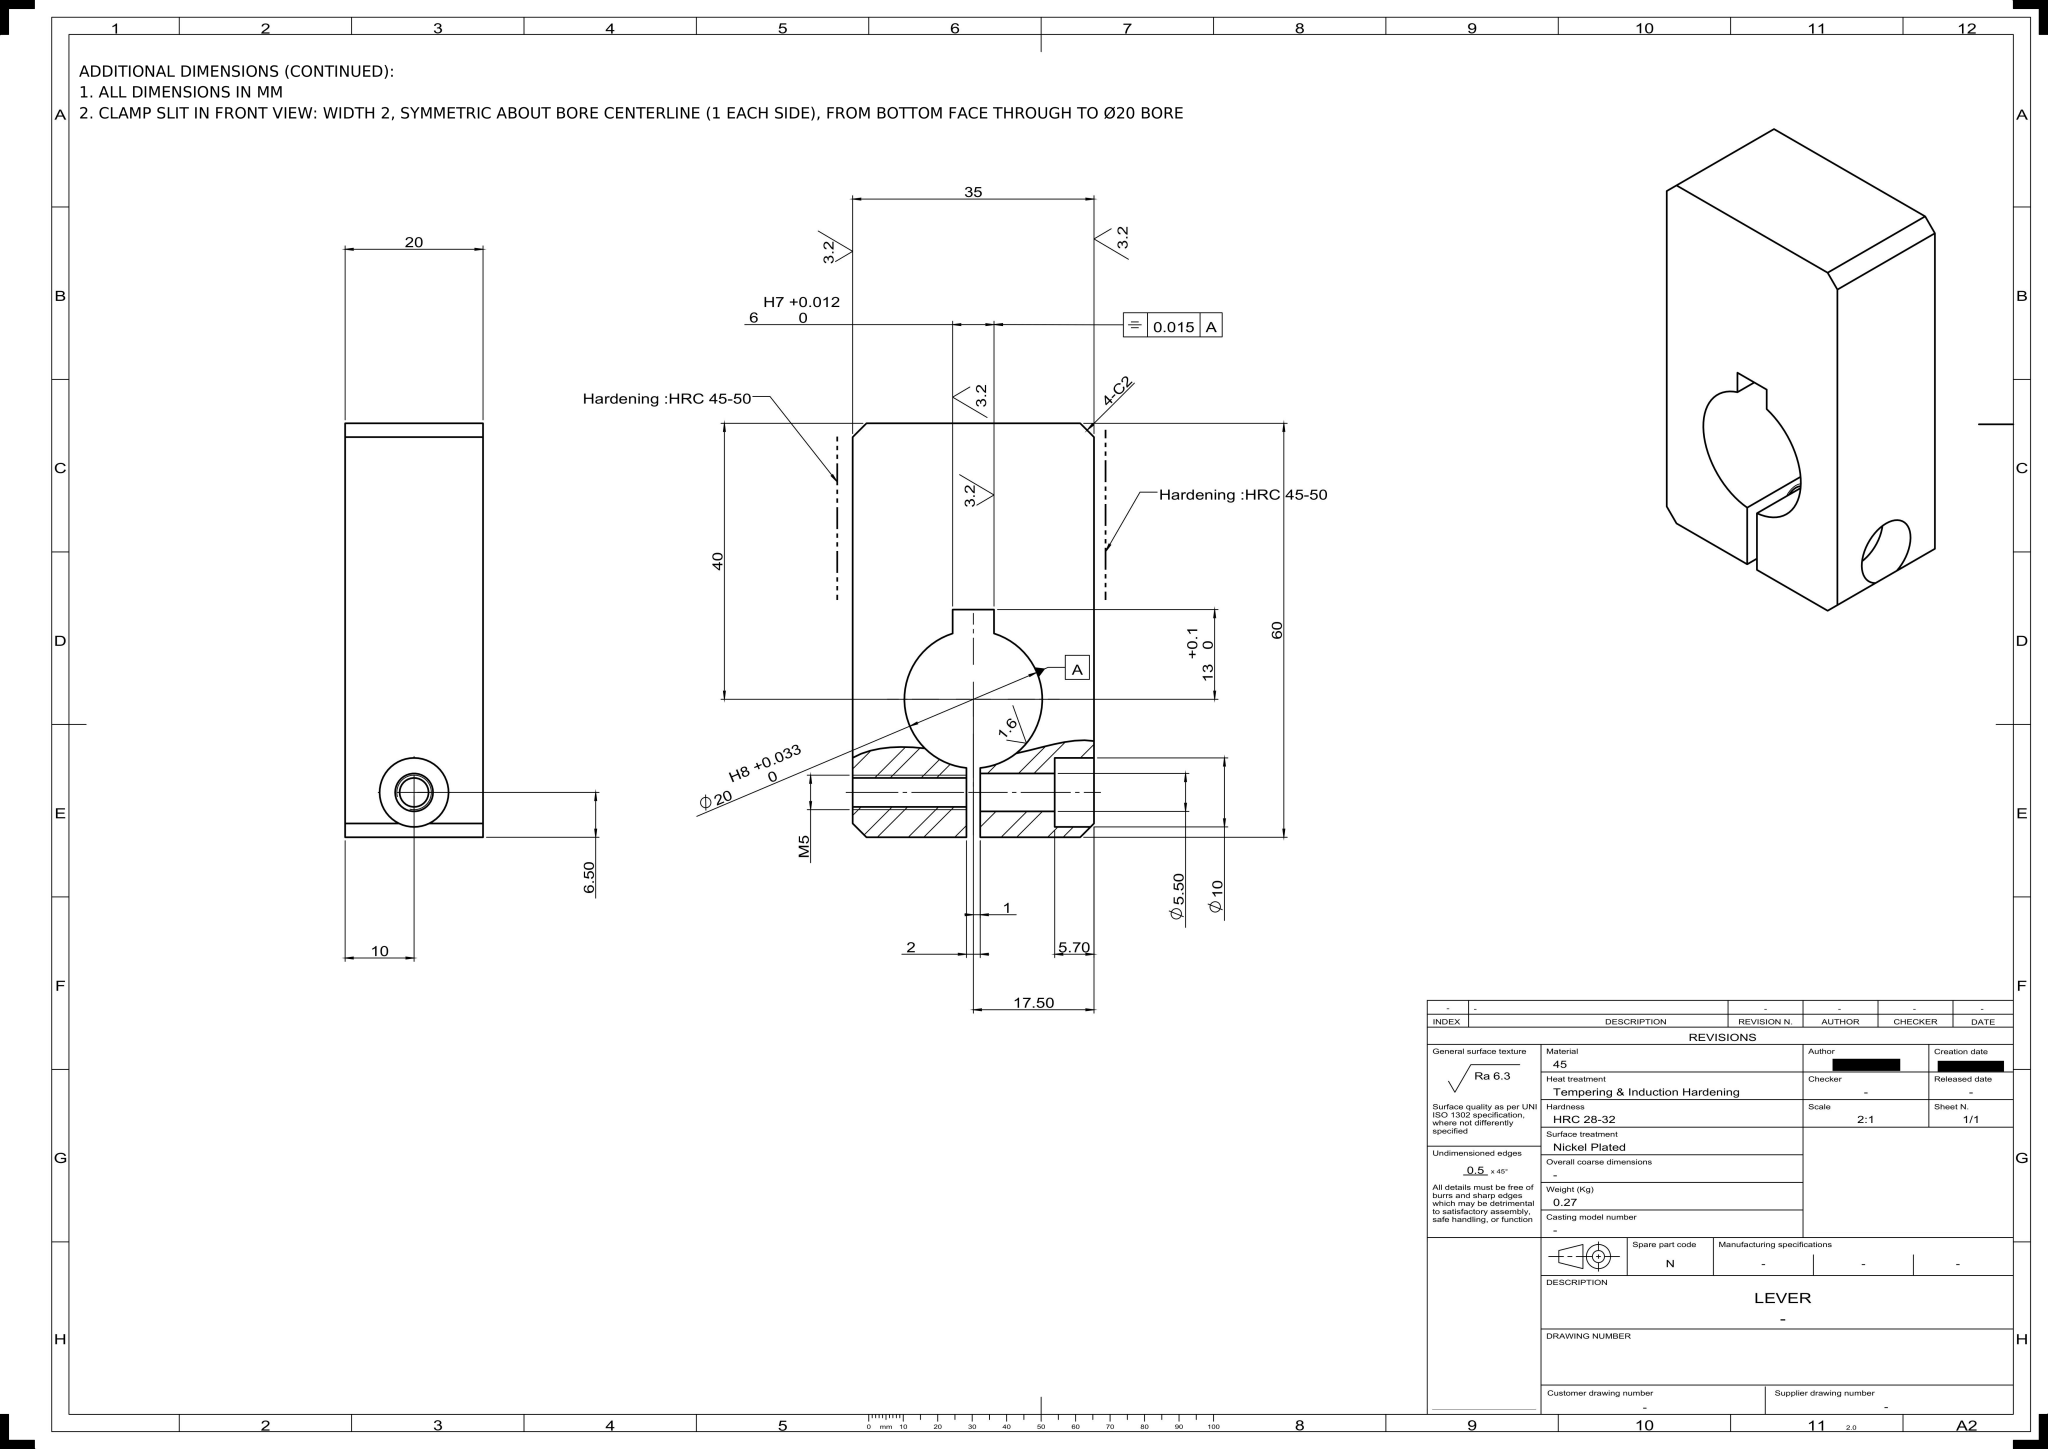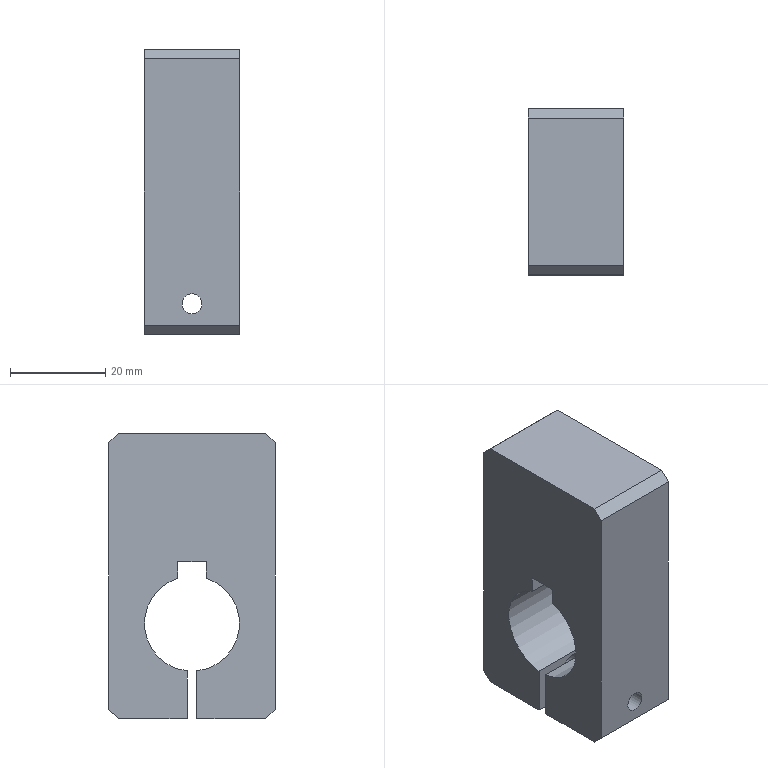Part | NX | mm | 1 solid | 22 faces | box 20 x 35 x 60 mm | volume 33845 mm3 | plane 17 | cylinder 5 | commonest cylinder face diameters 20 x2 5.5 x1 10 x1 4.2 x1
STEP:
#1=CARTESIAN_POINT('',(0.,0.,0.));
#2=DIRECTION('',(0.,0.,1.));
#3=DIRECTION('',(1.,0.,0.));
#4=AXIS2_PLACEMENT_3D('',#1,#2,#3);
#5=(LENGTH_UNIT()NAMED_UNIT(*)SI_UNIT(.MILLI.,.METRE.));
#6=UNCERTAINTY_MEASURE_WITH_UNIT(LENGTH_MEASURE(0.00002),#5,'','');
#7=(NAMED_UNIT(*)PLANE_ANGLE_UNIT()SI_UNIT($,.RADIAN.));
#8=PLANE_ANGLE_MEASURE_WITH_UNIT(PLANE_ANGLE_MEASURE(0.01745),#7);
#9=DIMENSIONAL_EXPONENTS(0.,0.,0.,0.,0.,0.,0.);
#10=(CONVERSION_BASED_UNIT('',#8)NAMED_UNIT(#9)PLANE_ANGLE_UNIT());
#11=(NAMED_UNIT(*)SI_UNIT($,.STERADIAN.)SOLID_ANGLE_UNIT());
#12=(GEOMETRIC_REPRESENTATION_CONTEXT(3)GLOBAL_UNCERTAINTY_ASSIGNED_CONTEXT((#6))GLOBAL_UNIT_ASSIGNED_CONTEXT((#5,#10,#11))REPRESENTATION_CONTEXT('',''));
#13=SHAPE_REPRESENTATION('',(#4),#12);
#14=CARTESIAN_POINT('',(10.,17.5,-18.));
#15=VERTEX_POINT('',#14);
#16=CARTESIAN_POINT('',(10.,17.5,38.));
#17=VERTEX_POINT('',#16);
#18=CARTESIAN_POINT('',(10.,17.5,-20.));
#19=DIRECTION('',(0.,0.,1.));
#20=VECTOR('',#19,1.);
#21=LINE('',#18,#20);
#22=EDGE_CURVE('',#15,#17,#21,.T.);
#23=ORIENTED_EDGE('',*,*,#22,.T.);
#24=CARTESIAN_POINT('',(10.,15.5,40.));
#25=VERTEX_POINT('',#24);
#26=CARTESIAN_POINT('',(10.,27.75,27.75));
#27=DIRECTION('',(0.,-0.7071,0.7071));
#28=VECTOR('',#27,1.);
#29=LINE('',#26,#28);
#30=EDGE_CURVE('',#17,#25,#29,.T.);
#31=ORIENTED_EDGE('',*,*,#30,.T.);
#32=CARTESIAN_POINT('',(10.,-15.5,40.));
#33=VERTEX_POINT('',#32);
#34=CARTESIAN_POINT('',(10.,17.5,40.));
#35=DIRECTION('',(0.,-1.,0.));
#36=VECTOR('',#35,1.);
#37=LINE('',#34,#36);
#38=EDGE_CURVE('',#25,#33,#37,.T.);
#39=ORIENTED_EDGE('',*,*,#38,.T.);
#40=CARTESIAN_POINT('',(10.,-17.5,38.));
#41=VERTEX_POINT('',#40);
#42=CARTESIAN_POINT('',(10.,-27.75,27.75));
#43=DIRECTION('',(0.,-0.7071,-0.7071));
#44=VECTOR('',#43,1.);
#45=LINE('',#42,#44);
#46=EDGE_CURVE('',#33,#41,#45,.T.);
#47=ORIENTED_EDGE('',*,*,#46,.T.);
#48=CARTESIAN_POINT('',(10.,-17.5,-18.));
#49=VERTEX_POINT('',#48);
#50=CARTESIAN_POINT('',(10.,-17.5,40.));
#51=DIRECTION('',(0.,0.,-1.));
#52=VECTOR('',#51,1.);
#53=LINE('',#50,#52);
#54=EDGE_CURVE('',#41,#49,#53,.T.);
#55=ORIENTED_EDGE('',*,*,#54,.T.);
#56=CARTESIAN_POINT('',(10.,-15.5,-20.));
#57=VERTEX_POINT('',#56);
#58=CARTESIAN_POINT('',(10.,-17.75,-17.75));
#59=DIRECTION('',(0.,0.7071,-0.7071));
#60=VECTOR('',#59,1.);
#61=LINE('',#58,#60);
#62=EDGE_CURVE('',#49,#57,#61,.T.);
#63=ORIENTED_EDGE('',*,*,#62,.T.);
#64=CARTESIAN_POINT('',(10.,-1.,-20.));
#65=VERTEX_POINT('',#64);
#66=CARTESIAN_POINT('',(10.,-17.5,-20.));
#67=DIRECTION('',(0.,1.,0.));
#68=VECTOR('',#67,1.);
#69=LINE('',#66,#68);
#70=EDGE_CURVE('',#57,#65,#69,.T.);
#71=ORIENTED_EDGE('',*,*,#70,.T.);
#72=CARTESIAN_POINT('',(10.,-1.,-9.95));
#73=VERTEX_POINT('',#72);
#74=CARTESIAN_POINT('',(10.,-1.,-20.));
#75=DIRECTION('',(0.,0.,1.));
#76=VECTOR('',#75,1.);
#77=LINE('',#74,#76);
#78=EDGE_CURVE('',#65,#73,#77,.T.);
#79=ORIENTED_EDGE('',*,*,#78,.T.);
#80=CARTESIAN_POINT('',(10.,-3.,9.539));
#81=VERTEX_POINT('',#80);
#82=CARTESIAN_POINT('',(10.,0.,0.));
#83=DIRECTION('',(-1.,0.,0.));
#84=DIRECTION('',(0.,0.,1.));
#85=AXIS2_PLACEMENT_3D('',#82,#83,#84);
#86=CIRCLE('',#85,10.);
#87=EDGE_CURVE('',#73,#81,#86,.T.);
#88=ORIENTED_EDGE('',*,*,#87,.T.);
#89=CARTESIAN_POINT('',(10.,-3.,13.));
#90=VERTEX_POINT('',#89);
#91=CARTESIAN_POINT('',(10.,-3.,0.));
#92=DIRECTION('',(0.,0.,1.));
#93=VECTOR('',#92,1.);
#94=LINE('',#91,#93);
#95=EDGE_CURVE('',#81,#90,#94,.T.);
#96=ORIENTED_EDGE('',*,*,#95,.T.);
#97=CARTESIAN_POINT('',(10.,3.,13.));
#98=VERTEX_POINT('',#97);
#99=CARTESIAN_POINT('',(10.,-3.,13.));
#100=DIRECTION('',(0.,1.,0.));
#101=VECTOR('',#100,1.);
#102=LINE('',#99,#101);
#103=EDGE_CURVE('',#90,#98,#102,.T.);
#104=ORIENTED_EDGE('',*,*,#103,.T.);
#105=CARTESIAN_POINT('',(10.,3.,9.539));
#106=VERTEX_POINT('',#105);
#107=CARTESIAN_POINT('',(10.,3.,13.));
#108=DIRECTION('',(0.,0.,-1.));
#109=VECTOR('',#108,1.);
#110=LINE('',#107,#109);
#111=EDGE_CURVE('',#98,#106,#110,.T.);
#112=ORIENTED_EDGE('',*,*,#111,.T.);
#113=CARTESIAN_POINT('',(10.,1.,-9.95));
#114=VERTEX_POINT('',#113);
#115=CARTESIAN_POINT('',(10.,0.,0.));
#116=DIRECTION('',(-1.,0.,0.));
#117=DIRECTION('',(0.,0.,1.));
#118=AXIS2_PLACEMENT_3D('',#115,#116,#117);
#119=CIRCLE('',#118,10.);
#120=EDGE_CURVE('',#106,#114,#119,.T.);
#121=ORIENTED_EDGE('',*,*,#120,.T.);
#122=CARTESIAN_POINT('',(10.,1.,-20.));
#123=VERTEX_POINT('',#122);
#124=CARTESIAN_POINT('',(10.,1.,0.));
#125=DIRECTION('',(0.,0.,-1.));
#126=VECTOR('',#125,1.);
#127=LINE('',#124,#126);
#128=EDGE_CURVE('',#114,#123,#127,.T.);
#129=ORIENTED_EDGE('',*,*,#128,.T.);
#130=CARTESIAN_POINT('',(10.,15.5,-20.));
#131=VERTEX_POINT('',#130);
#132=CARTESIAN_POINT('',(10.,1.,-20.));
#133=DIRECTION('',(0.,1.,0.));
#134=VECTOR('',#133,1.);
#135=LINE('',#132,#134);
#136=EDGE_CURVE('',#123,#131,#135,.T.);
#137=ORIENTED_EDGE('',*,*,#136,.T.);
#138=CARTESIAN_POINT('',(10.,17.75,-17.75));
#139=DIRECTION('',(0.,0.7071,0.7071));
#140=VECTOR('',#139,1.);
#141=LINE('',#138,#140);
#142=EDGE_CURVE('',#131,#15,#141,.T.);
#143=ORIENTED_EDGE('',*,*,#142,.T.);
#144=EDGE_LOOP('',(#23,#31,#39,#47,#55,#63,#71,#79,#88,#96,#104,#112,#121,#129,#137,#143));
#145=FACE_OUTER_BOUND('',#144,.T.);
#146=CARTESIAN_POINT('',(10.,0.,0.));
#147=DIRECTION('',(1.,0.,0.));
#148=DIRECTION('',(0.,0.,-1.));
#149=AXIS2_PLACEMENT_3D('',#146,#147,#148);
#150=PLANE('',#149);
#151=ADVANCED_FACE('',(#145),#150,.T.);
#152=CARTESIAN_POINT('',(0.,-17.5,-11.4));
#153=VERTEX_POINT('',#152);
#154=CARTESIAN_POINT('',(0.,-17.5,-13.5));
#155=DIRECTION('',(0.,1.,0.));
#156=DIRECTION('',(0.,0.,1.));
#157=AXIS2_PLACEMENT_3D('',#154,#155,#156);
#158=CIRCLE('',#157,2.1);
#159=EDGE_CURVE('',#153,#153,#158,.T.);
#160=ORIENTED_EDGE('',*,*,#159,.T.);
#161=EDGE_LOOP('',(#160));
#162=FACE_BOUND('',#161,.T.);
#163=ORIENTED_EDGE('',*,*,#54,.F.);
#164=CARTESIAN_POINT('',(-10.,-17.5,38.));
#165=VERTEX_POINT('',#164);
#166=CARTESIAN_POINT('',(10.,-17.5,38.));
#167=DIRECTION('',(-1.,0.,0.));
#168=VECTOR('',#167,1.);
#169=LINE('',#166,#168);
#170=EDGE_CURVE('',#41,#165,#169,.T.);
#171=ORIENTED_EDGE('',*,*,#170,.T.);
#172=CARTESIAN_POINT('',(-10.,-17.5,-18.));
#173=VERTEX_POINT('',#172);
#174=CARTESIAN_POINT('',(-10.,-17.5,40.));
#175=DIRECTION('',(0.,0.,-1.));
#176=VECTOR('',#175,1.);
#177=LINE('',#174,#176);
#178=EDGE_CURVE('',#165,#173,#177,.T.);
#179=ORIENTED_EDGE('',*,*,#178,.T.);
#180=CARTESIAN_POINT('',(10.,-17.5,-18.));
#181=DIRECTION('',(1.,0.,0.));
#182=VECTOR('',#181,1.);
#183=LINE('',#180,#182);
#184=EDGE_CURVE('',#173,#49,#183,.T.);
#185=ORIENTED_EDGE('',*,*,#184,.T.);
#186=EDGE_LOOP('',(#163,#171,#179,#185));
#187=FACE_BOUND('',#186,.T.);
#188=CARTESIAN_POINT('',(10.,-17.5,40.));
#189=DIRECTION('',(0.,1.,0.));
#190=DIRECTION('',(0.,0.,1.));
#191=AXIS2_PLACEMENT_3D('',#188,#189,#190);
#192=PLANE('',#191);
#193=ADVANCED_FACE('',(#162,#187),#192,.F.);
#194=ORIENTED_EDGE('',*,*,#70,.F.);
#195=CARTESIAN_POINT('',(-10.,-15.5,-20.));
#196=VERTEX_POINT('',#195);
#197=CARTESIAN_POINT('',(10.,-15.5,-20.));
#198=DIRECTION('',(-1.,0.,0.));
#199=VECTOR('',#198,1.);
#200=LINE('',#197,#199);
#201=EDGE_CURVE('',#57,#196,#200,.T.);
#202=ORIENTED_EDGE('',*,*,#201,.T.);
#203=CARTESIAN_POINT('',(-10.,-1.,-20.));
#204=VERTEX_POINT('',#203);
#205=CARTESIAN_POINT('',(-10.,-17.5,-20.));
#206=DIRECTION('',(0.,1.,0.));
#207=VECTOR('',#206,1.);
#208=LINE('',#205,#207);
#209=EDGE_CURVE('',#196,#204,#208,.T.);
#210=ORIENTED_EDGE('',*,*,#209,.T.);
#211=CARTESIAN_POINT('',(10.,-1.,-20.));
#212=DIRECTION('',(-1.,0.,0.));
#213=VECTOR('',#212,1.);
#214=LINE('',#211,#213);
#215=EDGE_CURVE('',#65,#204,#214,.T.);
#216=ORIENTED_EDGE('',*,*,#215,.F.);
#217=EDGE_LOOP('',(#194,#202,#210,#216));
#218=FACE_OUTER_BOUND('',#217,.T.);
#219=CARTESIAN_POINT('',(10.,-17.5,-20.));
#220=DIRECTION('',(0.,0.,1.));
#221=DIRECTION('',(1.,0.,0.));
#222=AXIS2_PLACEMENT_3D('',#219,#220,#221);
#223=PLANE('',#222);
#224=ADVANCED_FACE('',(#218),#223,.F.);
#225=CARTESIAN_POINT('',(0.,-1.,-15.6));
#226=VERTEX_POINT('',#225);
#227=CARTESIAN_POINT('',(0.,-1.,-13.5));
#228=DIRECTION('',(0.,-1.,0.));
#229=DIRECTION('',(0.,0.,-1.));
#230=AXIS2_PLACEMENT_3D('',#227,#228,#229);
#231=CIRCLE('',#230,2.1);
#232=EDGE_CURVE('',#226,#226,#231,.T.);
#233=ORIENTED_EDGE('',*,*,#232,.T.);
#234=EDGE_LOOP('',(#233));
#235=FACE_BOUND('',#234,.T.);
#236=CARTESIAN_POINT('',(-10.,-1.,-9.95));
#237=VERTEX_POINT('',#236);
#238=CARTESIAN_POINT('',(-10.,-1.,-20.));
#239=DIRECTION('',(0.,0.,1.));
#240=VECTOR('',#239,1.);
#241=LINE('',#238,#240);
#242=EDGE_CURVE('',#204,#237,#241,.T.);
#243=ORIENTED_EDGE('',*,*,#242,.T.);
#244=CARTESIAN_POINT('',(10.,-1.,-9.95));
#245=DIRECTION('',(1.,0.,0.));
#246=VECTOR('',#245,1.);
#247=LINE('',#244,#246);
#248=EDGE_CURVE('',#237,#73,#247,.T.);
#249=ORIENTED_EDGE('',*,*,#248,.T.);
#250=ORIENTED_EDGE('',*,*,#78,.F.);
#251=ORIENTED_EDGE('',*,*,#215,.T.);
#252=EDGE_LOOP('',(#243,#249,#250,#251));
#253=FACE_BOUND('',#252,.T.);
#254=CARTESIAN_POINT('',(10.,-1.,-20.));
#255=DIRECTION('',(0.,-1.,0.));
#256=DIRECTION('',(0.,0.,-1.));
#257=AXIS2_PLACEMENT_3D('',#254,#255,#256);
#258=PLANE('',#257);
#259=ADVANCED_FACE('',(#235,#253),#258,.F.);
#260=ORIENTED_EDGE('',*,*,#95,.F.);
#261=CARTESIAN_POINT('',(-10.,-3.,9.539));
#262=VERTEX_POINT('',#261);
#263=CARTESIAN_POINT('',(10.,-3.,9.539));
#264=DIRECTION('',(-1.,0.,0.));
#265=VECTOR('',#264,1.);
#266=LINE('',#263,#265);
#267=EDGE_CURVE('',#81,#262,#266,.T.);
#268=ORIENTED_EDGE('',*,*,#267,.T.);
#269=CARTESIAN_POINT('',(-10.,-3.,13.));
#270=VERTEX_POINT('',#269);
#271=CARTESIAN_POINT('',(-10.,-3.,0.));
#272=DIRECTION('',(0.,0.,1.));
#273=VECTOR('',#272,1.);
#274=LINE('',#271,#273);
#275=EDGE_CURVE('',#262,#270,#274,.T.);
#276=ORIENTED_EDGE('',*,*,#275,.T.);
#277=CARTESIAN_POINT('',(10.,-3.,13.));
#278=DIRECTION('',(-1.,0.,0.));
#279=VECTOR('',#278,1.);
#280=LINE('',#277,#279);
#281=EDGE_CURVE('',#90,#270,#280,.T.);
#282=ORIENTED_EDGE('',*,*,#281,.F.);
#283=EDGE_LOOP('',(#260,#268,#276,#282));
#284=FACE_OUTER_BOUND('',#283,.T.);
#285=CARTESIAN_POINT('',(10.,-3.,0.));
#286=DIRECTION('',(0.,-1.,0.));
#287=DIRECTION('',(0.,0.,-1.));
#288=AXIS2_PLACEMENT_3D('',#285,#286,#287);
#289=PLANE('',#288);
#290=ADVANCED_FACE('',(#284),#289,.F.);
#291=CARTESIAN_POINT('',(-10.,3.,13.));
#292=VERTEX_POINT('',#291);
#293=CARTESIAN_POINT('',(-10.,-3.,13.));
#294=DIRECTION('',(0.,1.,0.));
#295=VECTOR('',#294,1.);
#296=LINE('',#293,#295);
#297=EDGE_CURVE('',#270,#292,#296,.T.);
#298=ORIENTED_EDGE('',*,*,#297,.T.);
#299=CARTESIAN_POINT('',(10.,3.,13.));
#300=DIRECTION('',(-1.,0.,0.));
#301=VECTOR('',#300,1.);
#302=LINE('',#299,#301);
#303=EDGE_CURVE('',#98,#292,#302,.T.);
#304=ORIENTED_EDGE('',*,*,#303,.F.);
#305=ORIENTED_EDGE('',*,*,#103,.F.);
#306=ORIENTED_EDGE('',*,*,#281,.T.);
#307=EDGE_LOOP('',(#298,#304,#305,#306));
#308=FACE_OUTER_BOUND('',#307,.T.);
#309=CARTESIAN_POINT('',(10.,-3.,13.));
#310=DIRECTION('',(0.,0.,1.));
#311=DIRECTION('',(1.,0.,0.));
#312=AXIS2_PLACEMENT_3D('',#309,#310,#311);
#313=PLANE('',#312);
#314=ADVANCED_FACE('',(#308),#313,.F.);
#315=CARTESIAN_POINT('',(-10.,3.,9.539));
#316=VERTEX_POINT('',#315);
#317=CARTESIAN_POINT('',(-10.,3.,13.));
#318=DIRECTION('',(0.,0.,-1.));
#319=VECTOR('',#318,1.);
#320=LINE('',#317,#319);
#321=EDGE_CURVE('',#292,#316,#320,.T.);
#322=ORIENTED_EDGE('',*,*,#321,.T.);
#323=CARTESIAN_POINT('',(10.,3.,9.539));
#324=DIRECTION('',(1.,0.,0.));
#325=VECTOR('',#324,1.);
#326=LINE('',#323,#325);
#327=EDGE_CURVE('',#316,#106,#326,.T.);
#328=ORIENTED_EDGE('',*,*,#327,.T.);
#329=ORIENTED_EDGE('',*,*,#111,.F.);
#330=ORIENTED_EDGE('',*,*,#303,.T.);
#331=EDGE_LOOP('',(#322,#328,#329,#330));
#332=FACE_OUTER_BOUND('',#331,.T.);
#333=CARTESIAN_POINT('',(10.,3.,13.));
#334=DIRECTION('',(0.,1.,0.));
#335=DIRECTION('',(0.,0.,1.));
#336=AXIS2_PLACEMENT_3D('',#333,#334,#335);
#337=PLANE('',#336);
#338=ADVANCED_FACE('',(#332),#337,.F.);
#339=CARTESIAN_POINT('',(0.,1.,-10.75));
#340=VERTEX_POINT('',#339);
#341=CARTESIAN_POINT('',(0.,1.,-13.5));
#342=DIRECTION('',(0.,1.,0.));
#343=DIRECTION('',(0.,0.,1.));
#344=AXIS2_PLACEMENT_3D('',#341,#342,#343);
#345=CIRCLE('',#344,2.75);
#346=EDGE_CURVE('',#340,#340,#345,.T.);
#347=ORIENTED_EDGE('',*,*,#346,.T.);
#348=EDGE_LOOP('',(#347));
#349=FACE_BOUND('',#348,.T.);
#350=ORIENTED_EDGE('',*,*,#128,.F.);
#351=CARTESIAN_POINT('',(-10.,1.,-9.95));
#352=VERTEX_POINT('',#351);
#353=CARTESIAN_POINT('',(10.,1.,-9.95));
#354=DIRECTION('',(-1.,0.,0.));
#355=VECTOR('',#354,1.);
#356=LINE('',#353,#355);
#357=EDGE_CURVE('',#114,#352,#356,.T.);
#358=ORIENTED_EDGE('',*,*,#357,.T.);
#359=CARTESIAN_POINT('',(-10.,1.,-20.));
#360=VERTEX_POINT('',#359);
#361=CARTESIAN_POINT('',(-10.,1.,0.));
#362=DIRECTION('',(0.,0.,-1.));
#363=VECTOR('',#362,1.);
#364=LINE('',#361,#363);
#365=EDGE_CURVE('',#352,#360,#364,.T.);
#366=ORIENTED_EDGE('',*,*,#365,.T.);
#367=CARTESIAN_POINT('',(10.,1.,-20.));
#368=DIRECTION('',(-1.,0.,0.));
#369=VECTOR('',#368,1.);
#370=LINE('',#367,#369);
#371=EDGE_CURVE('',#123,#360,#370,.T.);
#372=ORIENTED_EDGE('',*,*,#371,.F.);
#373=EDGE_LOOP('',(#350,#358,#366,#372));
#374=FACE_BOUND('',#373,.T.);
#375=CARTESIAN_POINT('',(10.,1.,0.));
#376=DIRECTION('',(0.,1.,0.));
#377=DIRECTION('',(0.,0.,1.));
#378=AXIS2_PLACEMENT_3D('',#375,#376,#377);
#379=PLANE('',#378);
#380=ADVANCED_FACE('',(#349,#374),#379,.F.);
#381=CARTESIAN_POINT('',(-10.,15.5,-20.));
#382=VERTEX_POINT('',#381);
#383=CARTESIAN_POINT('',(-10.,1.,-20.));
#384=DIRECTION('',(0.,1.,0.));
#385=VECTOR('',#384,1.);
#386=LINE('',#383,#385);
#387=EDGE_CURVE('',#360,#382,#386,.T.);
#388=ORIENTED_EDGE('',*,*,#387,.T.);
#389=CARTESIAN_POINT('',(10.,15.5,-20.));
#390=DIRECTION('',(1.,0.,0.));
#391=VECTOR('',#390,1.);
#392=LINE('',#389,#391);
#393=EDGE_CURVE('',#382,#131,#392,.T.);
#394=ORIENTED_EDGE('',*,*,#393,.T.);
#395=ORIENTED_EDGE('',*,*,#136,.F.);
#396=ORIENTED_EDGE('',*,*,#371,.T.);
#397=EDGE_LOOP('',(#388,#394,#395,#396));
#398=FACE_OUTER_BOUND('',#397,.T.);
#399=CARTESIAN_POINT('',(10.,1.,-20.));
#400=DIRECTION('',(0.,0.,1.));
#401=DIRECTION('',(1.,0.,0.));
#402=AXIS2_PLACEMENT_3D('',#399,#400,#401);
#403=PLANE('',#402);
#404=ADVANCED_FACE('',(#398),#403,.F.);
#405=CARTESIAN_POINT('',(-10.,17.5,-18.));
#406=VERTEX_POINT('',#405);
#407=CARTESIAN_POINT('',(-10.,17.5,38.));
#408=VERTEX_POINT('',#407);
#409=CARTESIAN_POINT('',(-10.,17.5,-20.));
#410=DIRECTION('',(0.,0.,1.));
#411=VECTOR('',#410,1.);
#412=LINE('',#409,#411);
#413=EDGE_CURVE('',#406,#408,#412,.T.);
#414=ORIENTED_EDGE('',*,*,#413,.T.);
#415=CARTESIAN_POINT('',(10.,17.5,38.));
#416=DIRECTION('',(1.,0.,0.));
#417=VECTOR('',#416,1.);
#418=LINE('',#415,#417);
#419=EDGE_CURVE('',#408,#17,#418,.T.);
#420=ORIENTED_EDGE('',*,*,#419,.T.);
#421=ORIENTED_EDGE('',*,*,#22,.F.);
#422=CARTESIAN_POINT('',(2.179,17.5,-18.));
#423=VERTEX_POINT('',#422);
#424=CARTESIAN_POINT('',(10.,17.5,-18.));
#425=DIRECTION('',(-1.,0.,0.));
#426=VECTOR('',#425,1.);
#427=LINE('',#424,#426);
#428=EDGE_CURVE('',#15,#423,#427,.T.);
#429=ORIENTED_EDGE('',*,*,#428,.T.);
#430=CARTESIAN_POINT('',(-2.179,17.5,-18.));
#431=VERTEX_POINT('',#430);
#432=CARTESIAN_POINT('',(0.,17.5,-13.5));
#433=DIRECTION('',(0.,-1.,0.));
#434=DIRECTION('',(0.,0.,-1.));
#435=AXIS2_PLACEMENT_3D('',#432,#433,#434);
#436=CIRCLE('',#435,5.);
#437=EDGE_CURVE('',#423,#431,#436,.T.);
#438=ORIENTED_EDGE('',*,*,#437,.T.);
#439=CARTESIAN_POINT('',(10.,17.5,-18.));
#440=DIRECTION('',(-1.,0.,0.));
#441=VECTOR('',#440,1.);
#442=LINE('',#439,#441);
#443=EDGE_CURVE('',#431,#406,#442,.T.);
#444=ORIENTED_EDGE('',*,*,#443,.T.);
#445=EDGE_LOOP('',(#414,#420,#421,#429,#438,#444));
#446=FACE_OUTER_BOUND('',#445,.T.);
#447=CARTESIAN_POINT('',(10.,17.5,-20.));
#448=DIRECTION('',(0.,-1.,0.));
#449=DIRECTION('',(0.,0.,-1.));
#450=AXIS2_PLACEMENT_3D('',#447,#448,#449);
#451=PLANE('',#450);
#452=ADVANCED_FACE('',(#446),#451,.F.);
#453=ORIENTED_EDGE('',*,*,#38,.F.);
#454=CARTESIAN_POINT('',(-10.,15.5,40.));
#455=VERTEX_POINT('',#454);
#456=CARTESIAN_POINT('',(10.,15.5,40.));
#457=DIRECTION('',(-1.,0.,0.));
#458=VECTOR('',#457,1.);
#459=LINE('',#456,#458);
#460=EDGE_CURVE('',#25,#455,#459,.T.);
#461=ORIENTED_EDGE('',*,*,#460,.T.);
#462=CARTESIAN_POINT('',(-10.,-15.5,40.));
#463=VERTEX_POINT('',#462);
#464=CARTESIAN_POINT('',(-10.,17.5,40.));
#465=DIRECTION('',(0.,-1.,0.));
#466=VECTOR('',#465,1.);
#467=LINE('',#464,#466);
#468=EDGE_CURVE('',#455,#463,#467,.T.);
#469=ORIENTED_EDGE('',*,*,#468,.T.);
#470=CARTESIAN_POINT('',(10.,-15.5,40.));
#471=DIRECTION('',(1.,0.,0.));
#472=VECTOR('',#471,1.);
#473=LINE('',#470,#472);
#474=EDGE_CURVE('',#463,#33,#473,.T.);
#475=ORIENTED_EDGE('',*,*,#474,.T.);
#476=EDGE_LOOP('',(#453,#461,#469,#475));
#477=FACE_OUTER_BOUND('',#476,.T.);
#478=CARTESIAN_POINT('',(10.,17.5,40.));
#479=DIRECTION('',(0.,0.,-1.));
#480=DIRECTION('',(-1.,0.,0.));
#481=AXIS2_PLACEMENT_3D('',#478,#479,#480);
#482=PLANE('',#481);
#483=ADVANCED_FACE('',(#477),#482,.F.);
#484=ORIENTED_EDGE('',*,*,#468,.F.);
#485=CARTESIAN_POINT('',(-10.,15.5,40.));
#486=DIRECTION('',(0.,0.7071,-0.7071));
#487=VECTOR('',#486,1.);
#488=LINE('',#485,#487);
#489=EDGE_CURVE('',#455,#408,#488,.T.);
#490=ORIENTED_EDGE('',*,*,#489,.T.);
#491=ORIENTED_EDGE('',*,*,#413,.F.);
#492=CARTESIAN_POINT('',(-10.,17.5,-18.));
#493=DIRECTION('',(0.,-0.7071,-0.7071));
#494=VECTOR('',#493,1.);
#495=LINE('',#492,#494);
#496=EDGE_CURVE('',#406,#382,#495,.T.);
#497=ORIENTED_EDGE('',*,*,#496,.T.);
#498=ORIENTED_EDGE('',*,*,#387,.F.);
#499=ORIENTED_EDGE('',*,*,#365,.F.);
#500=CARTESIAN_POINT('',(-10.,0.,0.));
#501=DIRECTION('',(1.,0.,0.));
#502=DIRECTION('',(0.,0.,-1.));
#503=AXIS2_PLACEMENT_3D('',#500,#501,#502);
#504=CIRCLE('',#503,10.);
#505=EDGE_CURVE('',#352,#316,#504,.T.);
#506=ORIENTED_EDGE('',*,*,#505,.T.);
#507=ORIENTED_EDGE('',*,*,#321,.F.);
#508=ORIENTED_EDGE('',*,*,#297,.F.);
#509=ORIENTED_EDGE('',*,*,#275,.F.);
#510=CARTESIAN_POINT('',(-10.,0.,0.));
#511=DIRECTION('',(1.,0.,0.));
#512=DIRECTION('',(0.,0.,-1.));
#513=AXIS2_PLACEMENT_3D('',#510,#511,#512);
#514=CIRCLE('',#513,10.);
#515=EDGE_CURVE('',#262,#237,#514,.T.);
#516=ORIENTED_EDGE('',*,*,#515,.T.);
#517=ORIENTED_EDGE('',*,*,#242,.F.);
#518=ORIENTED_EDGE('',*,*,#209,.F.);
#519=CARTESIAN_POINT('',(-10.,-15.5,-20.));
#520=DIRECTION('',(0.,-0.7071,0.7071));
#521=VECTOR('',#520,1.);
#522=LINE('',#519,#521);
#523=EDGE_CURVE('',#196,#173,#522,.T.);
#524=ORIENTED_EDGE('',*,*,#523,.T.);
#525=ORIENTED_EDGE('',*,*,#178,.F.);
#526=CARTESIAN_POINT('',(-10.,-17.5,38.));
#527=DIRECTION('',(0.,0.7071,0.7071));
#528=VECTOR('',#527,1.);
#529=LINE('',#526,#528);
#530=EDGE_CURVE('',#165,#463,#529,.T.);
#531=ORIENTED_EDGE('',*,*,#530,.T.);
#532=EDGE_LOOP('',(#484,#490,#491,#497,#498,#499,#506,#507,#508,#509,#516,#517,#518,#524,#525,#531));
#533=FACE_OUTER_BOUND('',#532,.T.);
#534=CARTESIAN_POINT('',(-10.,0.,0.));
#535=DIRECTION('',(1.,0.,0.));
#536=DIRECTION('',(0.,0.,-1.));
#537=AXIS2_PLACEMENT_3D('',#534,#535,#536);
#538=PLANE('',#537);
#539=ADVANCED_FACE('',(#533),#538,.F.);
#540=ORIENTED_EDGE('',*,*,#515,.F.);
#541=ORIENTED_EDGE('',*,*,#267,.F.);
#542=ORIENTED_EDGE('',*,*,#87,.F.);
#543=ORIENTED_EDGE('',*,*,#248,.F.);
#544=EDGE_LOOP('',(#540,#541,#542,#543));
#545=FACE_OUTER_BOUND('',#544,.T.);
#546=CARTESIAN_POINT('',(10.,0.,0.));
#547=DIRECTION('',(-1.,0.,0.));
#548=DIRECTION('',(0.,0.,1.));
#549=AXIS2_PLACEMENT_3D('',#546,#547,#548);
#550=CYLINDRICAL_SURFACE('',#549,10.);
#551=ADVANCED_FACE('',(#545),#550,.F.);
#552=ORIENTED_EDGE('',*,*,#505,.F.);
#553=ORIENTED_EDGE('',*,*,#357,.F.);
#554=ORIENTED_EDGE('',*,*,#120,.F.);
#555=ORIENTED_EDGE('',*,*,#327,.F.);
#556=EDGE_LOOP('',(#552,#553,#554,#555));
#557=FACE_OUTER_BOUND('',#556,.T.);
#558=CARTESIAN_POINT('',(10.,0.,0.));
#559=DIRECTION('',(-1.,0.,0.));
#560=DIRECTION('',(0.,0.,1.));
#561=AXIS2_PLACEMENT_3D('',#558,#559,#560);
#562=CYLINDRICAL_SURFACE('',#561,10.);
#563=ADVANCED_FACE('',(#557),#562,.F.);
#564=CARTESIAN_POINT('',(0.,11.8,-16.25));
#565=VERTEX_POINT('',#564);
#566=CARTESIAN_POINT('',(0.,11.8,-13.5));
#567=DIRECTION('',(0.,1.,0.));
#568=DIRECTION('',(0.,0.,-1.));
#569=AXIS2_PLACEMENT_3D('',#566,#567,#568);
#570=CIRCLE('',#569,2.75);
#571=EDGE_CURVE('',#565,#565,#570,.T.);
#572=ORIENTED_EDGE('',*,*,#571,.T.);
#573=EDGE_LOOP('',(#572));
#574=FACE_BOUND('',#573,.T.);
#575=ORIENTED_EDGE('',*,*,#346,.F.);
#576=EDGE_LOOP('',(#575));
#577=FACE_BOUND('',#576,.T.);
#578=CARTESIAN_POINT('',(0.,-32.067,-13.5));
#579=DIRECTION('',(0.,-1.,0.));
#580=DIRECTION('',(0.,0.,-1.));
#581=AXIS2_PLACEMENT_3D('',#578,#579,#580);
#582=CYLINDRICAL_SURFACE('',#581,2.75);
#583=ADVANCED_FACE('',(#574,#577),#582,.F.);
#584=ORIENTED_EDGE('',*,*,#571,.F.);
#585=EDGE_LOOP('',(#584));
#586=FACE_BOUND('',#585,.T.);
#587=CARTESIAN_POINT('',(0.,11.8,-18.5));
#588=VERTEX_POINT('',#587);
#589=CARTESIAN_POINT('',(0.,11.8,-13.5));
#590=DIRECTION('',(0.,1.,0.));
#591=DIRECTION('',(0.,0.,-1.));
#592=AXIS2_PLACEMENT_3D('',#589,#590,#591);
#593=CIRCLE('',#592,5.);
#594=EDGE_CURVE('',#588,#588,#593,.T.);
#595=ORIENTED_EDGE('',*,*,#594,.T.);
#596=EDGE_LOOP('',(#595));
#597=FACE_BOUND('',#596,.T.);
#598=CARTESIAN_POINT('',(0.,11.8,-13.5));
#599=DIRECTION('',(0.,-1.,0.));
#600=DIRECTION('',(0.,0.,-1.));
#601=AXIS2_PLACEMENT_3D('',#598,#599,#600);
#602=PLANE('',#601);
#603=ADVANCED_FACE('',(#586,#597),#602,.F.);
#604=ORIENTED_EDGE('',*,*,#594,.F.);
#605=EDGE_LOOP('',(#604));
#606=FACE_BOUND('',#605,.T.);
#607=ORIENTED_EDGE('',*,*,#437,.F.);
#608=CARTESIAN_POINT('',(0.,22.,-13.5));
#609=DIRECTION('',(0.,0.7071,-0.7071));
#610=DIRECTION('',(0.,-0.7071,-0.7071));
#611=AXIS2_PLACEMENT_3D('',#608,#609,#610);
#612=ELLIPSE('',#611,7.071,5.);
#613=EDGE_CURVE('',#423,#431,#612,.T.);
#614=ORIENTED_EDGE('',*,*,#613,.T.);
#615=EDGE_LOOP('',(#607,#614));
#616=FACE_BOUND('',#615,.T.);
#617=CARTESIAN_POINT('',(0.,17.5,-13.5));
#618=DIRECTION('',(0.,-1.,0.));
#619=DIRECTION('',(0.,0.,-1.));
#620=AXIS2_PLACEMENT_3D('',#617,#618,#619);
#621=CYLINDRICAL_SURFACE('',#620,5.);
#622=ADVANCED_FACE('',(#606,#616),#621,.F.);
#623=ORIENTED_EDGE('',*,*,#232,.F.);
#624=EDGE_LOOP('',(#623));
#625=FACE_BOUND('',#624,.T.);
#626=ORIENTED_EDGE('',*,*,#159,.F.);
#627=EDGE_LOOP('',(#626));
#628=FACE_BOUND('',#627,.T.);
#629=CARTESIAN_POINT('',(0.,-1.,-13.5));
#630=DIRECTION('',(0.,-1.,0.));
#631=DIRECTION('',(0.,0.,-1.));
#632=AXIS2_PLACEMENT_3D('',#629,#630,#631);
#633=CYLINDRICAL_SURFACE('',#632,2.1);
#634=ADVANCED_FACE('',(#625,#628),#633,.F.);
#635=ORIENTED_EDGE('',*,*,#30,.F.);
#636=ORIENTED_EDGE('',*,*,#419,.F.);
#637=ORIENTED_EDGE('',*,*,#489,.F.);
#638=ORIENTED_EDGE('',*,*,#460,.F.);
#639=EDGE_LOOP('',(#635,#636,#637,#638));
#640=FACE_OUTER_BOUND('',#639,.T.);
#641=CARTESIAN_POINT('',(10.,15.5,40.));
#642=DIRECTION('',(0.,-0.7071,-0.7071));
#643=DIRECTION('',(-1.,0.,0.));
#644=AXIS2_PLACEMENT_3D('',#641,#642,#643);
#645=PLANE('',#644);
#646=ADVANCED_FACE('',(#640),#645,.F.);
#647=ORIENTED_EDGE('',*,*,#46,.F.);
#648=ORIENTED_EDGE('',*,*,#474,.F.);
#649=ORIENTED_EDGE('',*,*,#530,.F.);
#650=ORIENTED_EDGE('',*,*,#170,.F.);
#651=EDGE_LOOP('',(#647,#648,#649,#650));
#652=FACE_OUTER_BOUND('',#651,.T.);
#653=CARTESIAN_POINT('',(10.,-17.5,38.));
#654=DIRECTION('',(0.,0.7071,-0.7071));
#655=DIRECTION('',(-1.,0.,0.));
#656=AXIS2_PLACEMENT_3D('',#653,#654,#655);
#657=PLANE('',#656);
#658=ADVANCED_FACE('',(#652),#657,.F.);
#659=ORIENTED_EDGE('',*,*,#62,.F.);
#660=ORIENTED_EDGE('',*,*,#184,.F.);
#661=ORIENTED_EDGE('',*,*,#523,.F.);
#662=ORIENTED_EDGE('',*,*,#201,.F.);
#663=EDGE_LOOP('',(#659,#660,#661,#662));
#664=FACE_OUTER_BOUND('',#663,.T.);
#665=CARTESIAN_POINT('',(10.,-15.5,-20.));
#666=DIRECTION('',(0.,0.7071,0.7071));
#667=DIRECTION('',(-1.,0.,0.));
#668=AXIS2_PLACEMENT_3D('',#665,#666,#667);
#669=PLANE('',#668);
#670=ADVANCED_FACE('',(#664),#669,.F.);
#671=ORIENTED_EDGE('',*,*,#142,.F.);
#672=ORIENTED_EDGE('',*,*,#393,.F.);
#673=ORIENTED_EDGE('',*,*,#496,.F.);
#674=ORIENTED_EDGE('',*,*,#443,.F.);
#675=ORIENTED_EDGE('',*,*,#613,.F.);
#676=ORIENTED_EDGE('',*,*,#428,.F.);
#677=EDGE_LOOP('',(#671,#672,#673,#674,#675,#676));
#678=FACE_OUTER_BOUND('',#677,.T.);
#679=CARTESIAN_POINT('',(10.,17.5,-18.));
#680=DIRECTION('',(0.,-0.7071,0.7071));
#681=DIRECTION('',(-1.,0.,0.));
#682=AXIS2_PLACEMENT_3D('',#679,#680,#681);
#683=PLANE('',#682);
#684=ADVANCED_FACE('',(#678),#683,.F.);
#685=CLOSED_SHELL('',(#151,#193,#224,#259,#290,#314,#338,#380,#404,#452,#483,#539,#551,#563,#583,#603,#622,#634,#646,#658,#670,#684));
#686=MANIFOLD_SOLID_BREP('',#685);
#687=ADVANCED_BREP_SHAPE_REPRESENTATION('',(#686),#12);
#688=SHAPE_REPRESENTATION_RELATIONSHIP('','',#13,#687);
#689=PRESENTATION_LAYER_ASSIGNMENT('','',(#686));
#690=COLOUR_RGB('',0.4,0.8,1.);
#691=FILL_AREA_STYLE_COLOUR('',#690);
#692=FILL_AREA_STYLE('',(#691));
#693=SURFACE_STYLE_FILL_AREA(#692);
#694=SURFACE_SIDE_STYLE('',(#693));
#695=SURFACE_STYLE_USAGE(.BOTH.,#694);
#696=PRESENTATION_STYLE_ASSIGNMENT((#695));
#697=STYLED_ITEM('',(#696),#686);
#698=MECHANICAL_DESIGN_GEOMETRIC_PRESENTATION_REPRESENTATION('',(#697),#12);